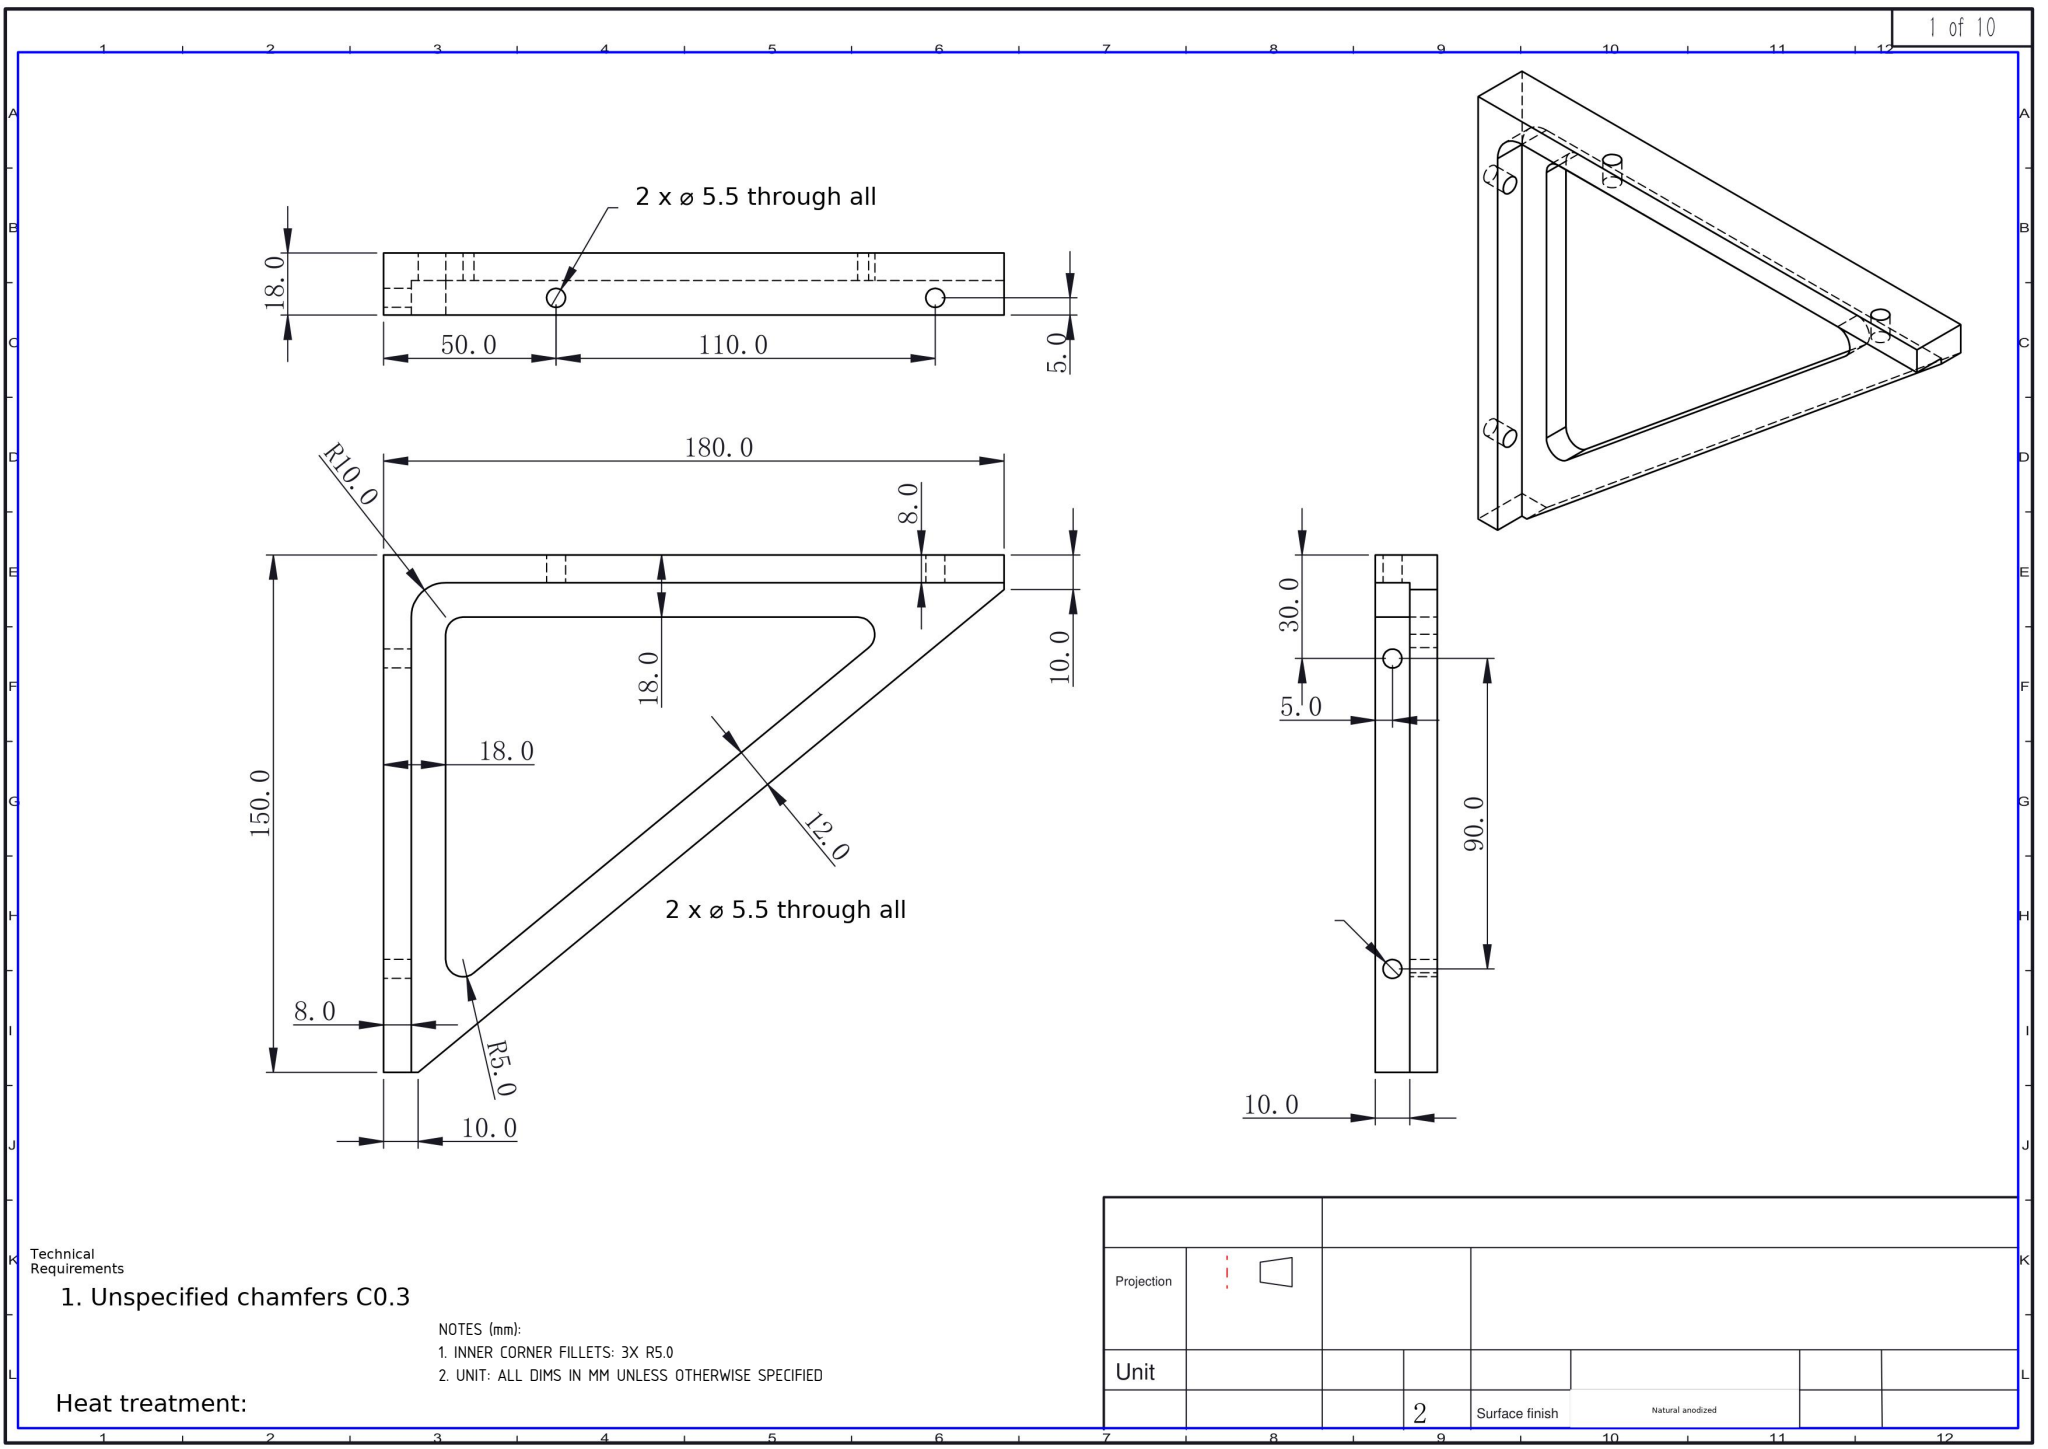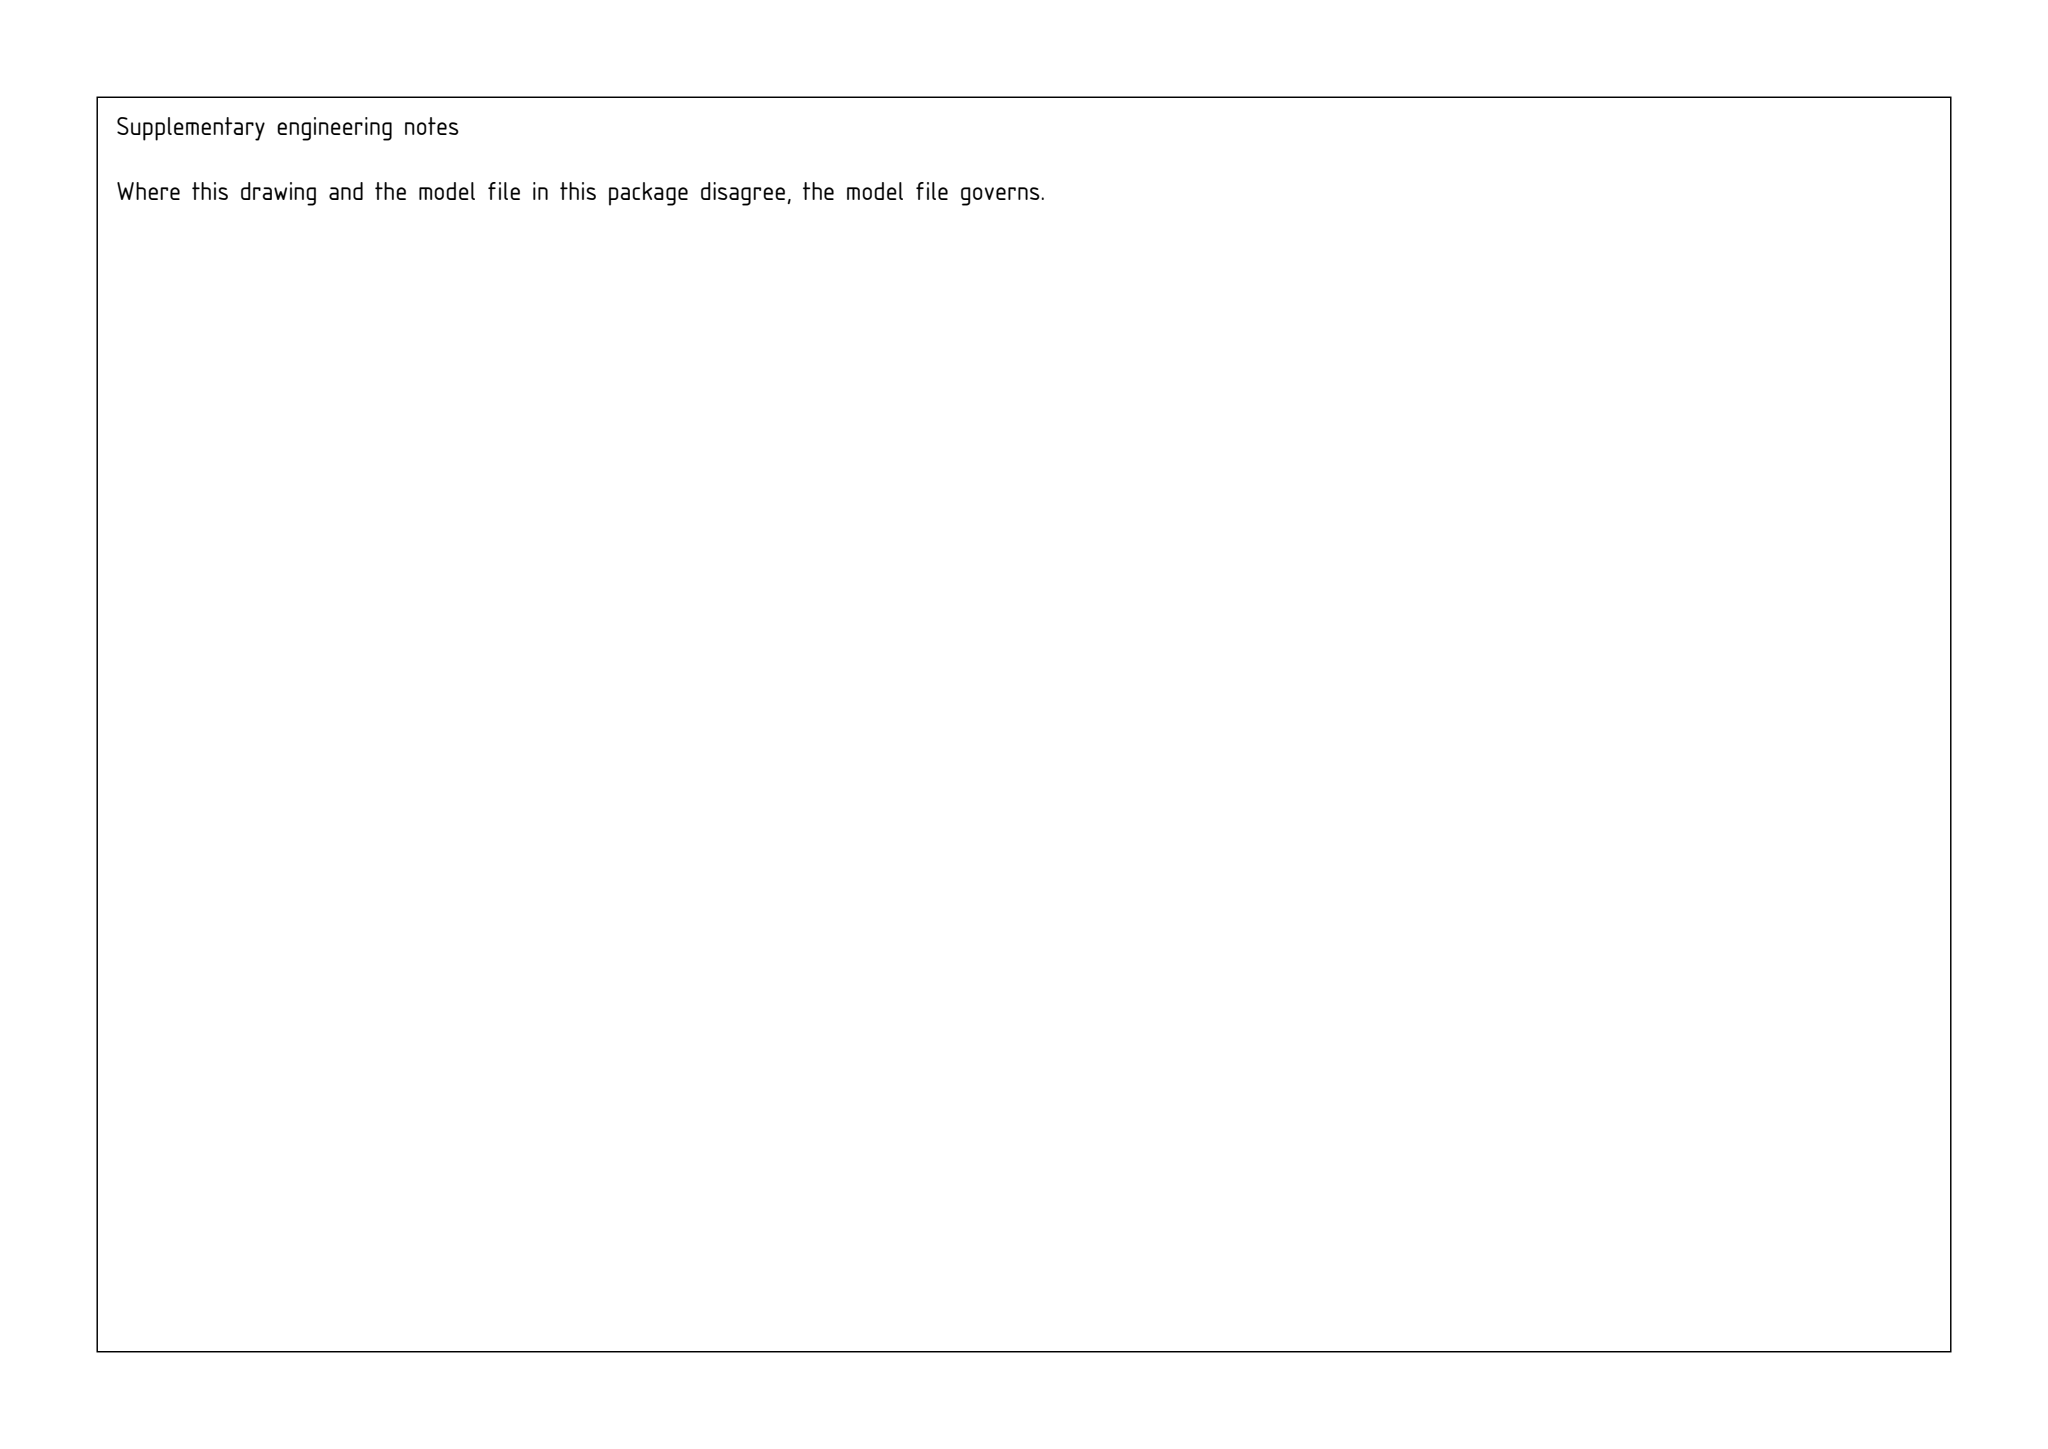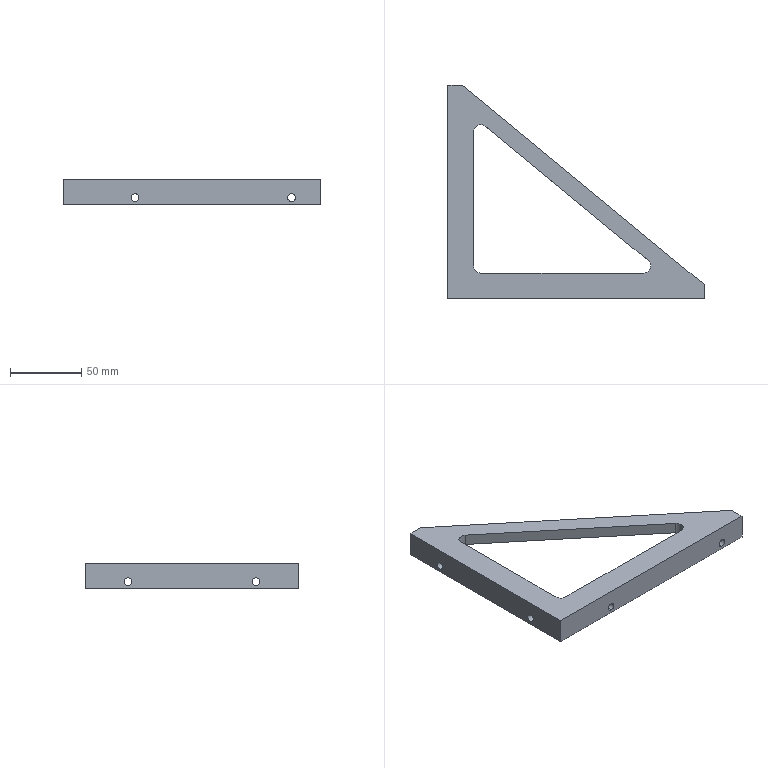Part | SolidWorks | mm | 1 solid | 25 faces | box 180 x 150 x 18 mm | volume 87939 mm3 | plane 13 | cylinder 12 | commonest cylinder face diameters 5.5 x8 10 x3 20 x1
Drawing notes:
INNER CORNER FILLETS: 3X R5.0 | from the solid: Three Ø10 z-axis cyls at (23,23), (23,117.27), (137.47,23) = R5.0 each
UNIT: ALL DIMS IN MM UNLESS OTHERWISE SPECIFIED | from the solid: STEP model bbox 180.0 x 150.0 x 18.0 mm matches drawing values
build123d program:
from build123d import *

# Parameters (mm, degrees)
BOSS_EXTRUDE1_DEPTH  = 18
CUT_EXTRUDE2_DEPTH   = 10
CUT_EXTRUDE3_DEPTH   = 235.521
M5_CLEARANCE_HOLE1_D = 5.5
M5_CLEARANCE_HOLE2_D = 5.5


with BuildPart() as part:
    # Sketch1 → Boss-Extrude1 (new body)
    with BuildSketch(Plane.XY):
        Polygon((10, 150), (180, 10), (180, 0), (0, 0), (0, 150), align=None)
    extrude(amount=BOSS_EXTRUDE1_DEPTH)

    # Sketch10 → Cut-Extrude2 (cut)
    with BuildSketch(Plane(origin=(0, 0, 0), x_dir=(-1, 0, 0), z_dir=(0, 0, -1))):
        with BuildLine():
            Line((-8, 150), (-180, 150))
            Line((-180, 150), (-180, 8))
            Line((-180, 8), (-18, 8))
            ThreePointArc((-18, 8), (-10.929, 10.929), (-8, 18))
            Line((-8, 18), (-8, 150))
        make_face()
    extrude(amount=-CUT_EXTRUDE2_DEPTH, mode=Mode.SUBTRACT)

    # Sketch11 → Cut-Extrude3 (cut, through all)
    with BuildSketch(Plane(origin=(0, 0, 10), x_dir=(-1, 0, 0), z_dir=(0, 0, -1))):
        with BuildLine():
            Line((-18, 23), (-18, 117.271))
            ThreePointArc((-18, 117.271), (-20.866, 121.793), (-26.179, 121.131))
            Line((-26.179, 121.131), (-140.651, 26.86))
            ThreePointArc((-140.651, 26.86), (-142.179, 21.312), (-137.472, 18))
            Line((-137.472, 18), (-23, 18))
            ThreePointArc((-23, 18), (-19.464, 19.464), (-18, 23))
        make_face()
    extrude(amount=-CUT_EXTRUDE3_DEPTH, mode=Mode.SUBTRACT)

    # M5 Clearance Hole1 (through all)
    with Locations(Plane(origin=(8, 0, 0), x_dir=(0, 0, -1), z_dir=(1, 0, 0))):
        with Locations((-5, 30), (-5, 120)):
            Hole(M5_CLEARANCE_HOLE1_D / 2)

    # M5 Clearance Hole2 (through all)
    with Locations(Plane(origin=(0, 8, 0), x_dir=(1, 0, 0), z_dir=(0, 1, 0))):
        with Locations((50, -5), (160, -5)):
            Hole(M5_CLEARANCE_HOLE2_D / 2)


solid = part.part
STEP:
#1=CARTESIAN_POINT('',(50.,-0.,2.25));
#2=VERTEX_POINT('',#1);
#3=CARTESIAN_POINT('',(50.,-0.,7.75));
#4=VERTEX_POINT('',#3);
#5=CARTESIAN_POINT('',(50.,-0.,5.));
#6=DIRECTION('',(0.,1.,0.));
#7=DIRECTION('',(0.,0.,1.));
#8=AXIS2_PLACEMENT_3D('',#5,#6,#7);
#9=CIRCLE('',#8,2.75);
#10=EDGE_CURVE('',#2,#4,#9,.T.);
#11=ORIENTED_EDGE('',*,*,#10,.F.);
#12=CARTESIAN_POINT('',(50.,8.,2.25));
#13=VERTEX_POINT('',#12);
#14=CARTESIAN_POINT('',(50.,8.,2.25));
#15=DIRECTION('',(0.,1.,0.));
#16=VECTOR('',#15,1000.);
#17=LINE('',#14,#16);
#18=EDGE_CURVE('',#2,#13,#17,.T.);
#19=ORIENTED_EDGE('',*,*,#18,.T.);
#20=CARTESIAN_POINT('',(50.,8.,7.75));
#21=VERTEX_POINT('',#20);
#22=CARTESIAN_POINT('',(50.,8.,5.));
#23=DIRECTION('',(0.,1.,0.));
#24=DIRECTION('',(0.,0.,1.));
#25=AXIS2_PLACEMENT_3D('',#22,#23,#24);
#26=CIRCLE('',#25,2.75);
#27=EDGE_CURVE('',#13,#21,#26,.T.);
#28=ORIENTED_EDGE('',*,*,#27,.T.);
#29=CARTESIAN_POINT('',(50.,8.,7.75));
#30=DIRECTION('',(0.,1.,0.));
#31=VECTOR('',#30,1000.);
#32=LINE('',#29,#31);
#33=EDGE_CURVE('',#4,#21,#32,.T.);
#34=ORIENTED_EDGE('',*,*,#33,.F.);
#35=EDGE_LOOP('',(#11,#19,#28,#34));
#36=FACE_OUTER_BOUND('',#35,.T.);
#37=CARTESIAN_POINT('',(50.,8.,5.));
#38=DIRECTION('',(0.,1.,0.));
#39=DIRECTION('',(0.,0.,1.));
#40=AXIS2_PLACEMENT_3D('',#37,#38,#39);
#41=CYLINDRICAL_SURFACE('',#40,2.75);
#42=ADVANCED_FACE('',(#36),#41,.F.);
#43=CARTESIAN_POINT('',(160.,-0.,2.25));
#44=VERTEX_POINT('',#43);
#45=CARTESIAN_POINT('',(160.,-0.,7.75));
#46=VERTEX_POINT('',#45);
#47=CARTESIAN_POINT('',(160.,-0.,5.));
#48=DIRECTION('',(0.,1.,0.));
#49=DIRECTION('',(0.,0.,1.));
#50=AXIS2_PLACEMENT_3D('',#47,#48,#49);
#51=CIRCLE('',#50,2.75);
#52=EDGE_CURVE('',#44,#46,#51,.T.);
#53=ORIENTED_EDGE('',*,*,#52,.F.);
#54=CARTESIAN_POINT('',(160.,8.,2.25));
#55=VERTEX_POINT('',#54);
#56=CARTESIAN_POINT('',(160.,8.,2.25));
#57=DIRECTION('',(0.,1.,0.));
#58=VECTOR('',#57,1000.);
#59=LINE('',#56,#58);
#60=EDGE_CURVE('',#44,#55,#59,.T.);
#61=ORIENTED_EDGE('',*,*,#60,.T.);
#62=CARTESIAN_POINT('',(160.,8.,7.75));
#63=VERTEX_POINT('',#62);
#64=CARTESIAN_POINT('',(160.,8.,5.));
#65=DIRECTION('',(0.,1.,0.));
#66=DIRECTION('',(0.,0.,1.));
#67=AXIS2_PLACEMENT_3D('',#64,#65,#66);
#68=CIRCLE('',#67,2.75);
#69=EDGE_CURVE('',#55,#63,#68,.T.);
#70=ORIENTED_EDGE('',*,*,#69,.T.);
#71=CARTESIAN_POINT('',(160.,8.,7.75));
#72=DIRECTION('',(0.,1.,0.));
#73=VECTOR('',#72,1000.);
#74=LINE('',#71,#73);
#75=EDGE_CURVE('',#46,#63,#74,.T.);
#76=ORIENTED_EDGE('',*,*,#75,.F.);
#77=EDGE_LOOP('',(#53,#61,#70,#76));
#78=FACE_OUTER_BOUND('',#77,.T.);
#79=CARTESIAN_POINT('',(160.,8.,5.));
#80=DIRECTION('',(0.,1.,0.));
#81=DIRECTION('',(0.,0.,1.));
#82=AXIS2_PLACEMENT_3D('',#79,#80,#81);
#83=CYLINDRICAL_SURFACE('',#82,2.75);
#84=ADVANCED_FACE('',(#78),#83,.F.);
#85=CARTESIAN_POINT('',(-0.,30.,7.75));
#86=VERTEX_POINT('',#85);
#87=CARTESIAN_POINT('',(-0.,30.,2.25));
#88=VERTEX_POINT('',#87);
#89=CARTESIAN_POINT('',(-0.,30.,5.));
#90=DIRECTION('',(1.,0.,0.));
#91=DIRECTION('',(0.,0.,-1.));
#92=AXIS2_PLACEMENT_3D('',#89,#90,#91);
#93=CIRCLE('',#92,2.75);
#94=EDGE_CURVE('',#86,#88,#93,.T.);
#95=ORIENTED_EDGE('',*,*,#94,.F.);
#96=CARTESIAN_POINT('',(8.,30.,7.75));
#97=VERTEX_POINT('',#96);
#98=CARTESIAN_POINT('',(8.,30.,7.75));
#99=DIRECTION('',(1.,0.,0.));
#100=VECTOR('',#99,1000.);
#101=LINE('',#98,#100);
#102=EDGE_CURVE('',#86,#97,#101,.T.);
#103=ORIENTED_EDGE('',*,*,#102,.T.);
#104=CARTESIAN_POINT('',(8.,30.,2.25));
#105=VERTEX_POINT('',#104);
#106=CARTESIAN_POINT('',(8.,30.,5.));
#107=DIRECTION('',(1.,0.,0.));
#108=DIRECTION('',(0.,0.,-1.));
#109=AXIS2_PLACEMENT_3D('',#106,#107,#108);
#110=CIRCLE('',#109,2.75);
#111=EDGE_CURVE('',#97,#105,#110,.T.);
#112=ORIENTED_EDGE('',*,*,#111,.T.);
#113=CARTESIAN_POINT('',(8.,30.,2.25));
#114=DIRECTION('',(1.,0.,0.));
#115=VECTOR('',#114,1000.);
#116=LINE('',#113,#115);
#117=EDGE_CURVE('',#88,#105,#116,.T.);
#118=ORIENTED_EDGE('',*,*,#117,.F.);
#119=EDGE_LOOP('',(#95,#103,#112,#118));
#120=FACE_OUTER_BOUND('',#119,.T.);
#121=CARTESIAN_POINT('',(8.,30.,5.));
#122=DIRECTION('',(1.,0.,0.));
#123=DIRECTION('',(0.,0.,-1.));
#124=AXIS2_PLACEMENT_3D('',#121,#122,#123);
#125=CYLINDRICAL_SURFACE('',#124,2.75);
#126=ADVANCED_FACE('',(#120),#125,.F.);
#127=CARTESIAN_POINT('',(-0.,120.,7.75));
#128=VERTEX_POINT('',#127);
#129=CARTESIAN_POINT('',(-0.,120.,2.25));
#130=VERTEX_POINT('',#129);
#131=CARTESIAN_POINT('',(-0.,120.,5.));
#132=DIRECTION('',(1.,0.,0.));
#133=DIRECTION('',(0.,0.,-1.));
#134=AXIS2_PLACEMENT_3D('',#131,#132,#133);
#135=CIRCLE('',#134,2.75);
#136=EDGE_CURVE('',#128,#130,#135,.T.);
#137=ORIENTED_EDGE('',*,*,#136,.F.);
#138=CARTESIAN_POINT('',(8.,120.,7.75));
#139=VERTEX_POINT('',#138);
#140=CARTESIAN_POINT('',(8.,120.,7.75));
#141=DIRECTION('',(1.,0.,0.));
#142=VECTOR('',#141,1000.);
#143=LINE('',#140,#142);
#144=EDGE_CURVE('',#128,#139,#143,.T.);
#145=ORIENTED_EDGE('',*,*,#144,.T.);
#146=CARTESIAN_POINT('',(8.,120.,2.25));
#147=VERTEX_POINT('',#146);
#148=CARTESIAN_POINT('',(8.,120.,5.));
#149=DIRECTION('',(1.,0.,0.));
#150=DIRECTION('',(0.,0.,-1.));
#151=AXIS2_PLACEMENT_3D('',#148,#149,#150);
#152=CIRCLE('',#151,2.75);
#153=EDGE_CURVE('',#139,#147,#152,.T.);
#154=ORIENTED_EDGE('',*,*,#153,.T.);
#155=CARTESIAN_POINT('',(8.,120.,2.25));
#156=DIRECTION('',(1.,0.,0.));
#157=VECTOR('',#156,1000.);
#158=LINE('',#155,#157);
#159=EDGE_CURVE('',#130,#147,#158,.T.);
#160=ORIENTED_EDGE('',*,*,#159,.F.);
#161=EDGE_LOOP('',(#137,#145,#154,#160));
#162=FACE_OUTER_BOUND('',#161,.T.);
#163=CARTESIAN_POINT('',(8.,120.,5.));
#164=DIRECTION('',(1.,0.,0.));
#165=DIRECTION('',(0.,0.,-1.));
#166=AXIS2_PLACEMENT_3D('',#163,#164,#165);
#167=CYLINDRICAL_SURFACE('',#166,2.75);
#168=ADVANCED_FACE('',(#162),#167,.F.);
#169=CARTESIAN_POINT('',(-0.,30.,5.));
#170=DIRECTION('',(1.,0.,0.));
#171=DIRECTION('',(0.,0.,-1.));
#172=AXIS2_PLACEMENT_3D('',#169,#170,#171);
#173=CIRCLE('',#172,2.75);
#174=EDGE_CURVE('',#88,#86,#173,.T.);
#175=ORIENTED_EDGE('',*,*,#174,.T.);
#176=ORIENTED_EDGE('',*,*,#94,.T.);
#177=EDGE_LOOP('',(#175,#176));
#178=FACE_BOUND('',#177,.T.);
#179=CARTESIAN_POINT('',(-0.,120.,5.));
#180=DIRECTION('',(1.,0.,0.));
#181=DIRECTION('',(0.,0.,-1.));
#182=AXIS2_PLACEMENT_3D('',#179,#180,#181);
#183=CIRCLE('',#182,2.75);
#184=EDGE_CURVE('',#130,#128,#183,.T.);
#185=ORIENTED_EDGE('',*,*,#184,.T.);
#186=ORIENTED_EDGE('',*,*,#136,.T.);
#187=EDGE_LOOP('',(#185,#186));
#188=FACE_BOUND('',#187,.T.);
#189=CARTESIAN_POINT('',(0.,150.,0.));
#190=VERTEX_POINT('',#189);
#191=CARTESIAN_POINT('',(0.,0.,0.));
#192=VERTEX_POINT('',#191);
#193=CARTESIAN_POINT('',(0.,0.,0.));
#194=DIRECTION('',(0.,-1.,0.));
#195=VECTOR('',#194,1000.);
#196=LINE('',#193,#195);
#197=EDGE_CURVE('',#190,#192,#196,.T.);
#198=ORIENTED_EDGE('',*,*,#197,.T.);
#199=CARTESIAN_POINT('',(0.,0.,18.));
#200=VERTEX_POINT('',#199);
#201=CARTESIAN_POINT('',(0.,0.,18.));
#202=DIRECTION('',(0.,0.,-1.));
#203=VECTOR('',#202,1000.);
#204=LINE('',#201,#203);
#205=EDGE_CURVE('',#200,#192,#204,.T.);
#206=ORIENTED_EDGE('',*,*,#205,.F.);
#207=CARTESIAN_POINT('',(0.,150.,18.));
#208=VERTEX_POINT('',#207);
#209=CARTESIAN_POINT('',(0.,0.,18.));
#210=DIRECTION('',(0.,-1.,0.));
#211=VECTOR('',#210,1000.);
#212=LINE('',#209,#211);
#213=EDGE_CURVE('',#208,#200,#212,.T.);
#214=ORIENTED_EDGE('',*,*,#213,.F.);
#215=CARTESIAN_POINT('',(0.,150.,18.));
#216=DIRECTION('',(0.,0.,-1.));
#217=VECTOR('',#216,1000.);
#218=LINE('',#215,#217);
#219=EDGE_CURVE('',#208,#190,#218,.T.);
#220=ORIENTED_EDGE('',*,*,#219,.T.);
#221=EDGE_LOOP('',(#198,#206,#214,#220));
#222=FACE_OUTER_BOUND('',#221,.T.);
#223=CARTESIAN_POINT('',(0.,0.,18.));
#224=DIRECTION('',(1.,0.,0.));
#225=DIRECTION('',(0.,0.,-1.));
#226=AXIS2_PLACEMENT_3D('',#223,#224,#225);
#227=PLANE('',#226);
#228=ADVANCED_FACE('',(#178,#188,#222),#227,.F.);
#229=CARTESIAN_POINT('',(50.,-0.,5.));
#230=DIRECTION('',(0.,1.,0.));
#231=DIRECTION('',(0.,0.,1.));
#232=AXIS2_PLACEMENT_3D('',#229,#230,#231);
#233=CIRCLE('',#232,2.75);
#234=EDGE_CURVE('',#4,#2,#233,.T.);
#235=ORIENTED_EDGE('',*,*,#234,.T.);
#236=ORIENTED_EDGE('',*,*,#10,.T.);
#237=EDGE_LOOP('',(#235,#236));
#238=FACE_BOUND('',#237,.T.);
#239=CARTESIAN_POINT('',(160.,-0.,5.));
#240=DIRECTION('',(0.,1.,0.));
#241=DIRECTION('',(0.,0.,1.));
#242=AXIS2_PLACEMENT_3D('',#239,#240,#241);
#243=CIRCLE('',#242,2.75);
#244=EDGE_CURVE('',#46,#44,#243,.T.);
#245=ORIENTED_EDGE('',*,*,#244,.T.);
#246=ORIENTED_EDGE('',*,*,#52,.T.);
#247=EDGE_LOOP('',(#245,#246));
#248=FACE_BOUND('',#247,.T.);
#249=CARTESIAN_POINT('',(180.,0.,0.));
#250=VERTEX_POINT('',#249);
#251=CARTESIAN_POINT('',(0.,0.,0.));
#252=DIRECTION('',(1.,0.,0.));
#253=VECTOR('',#252,1000.);
#254=LINE('',#251,#253);
#255=EDGE_CURVE('',#192,#250,#254,.T.);
#256=ORIENTED_EDGE('',*,*,#255,.T.);
#257=CARTESIAN_POINT('',(180.,0.,18.));
#258=VERTEX_POINT('',#257);
#259=CARTESIAN_POINT('',(180.,0.,18.));
#260=DIRECTION('',(0.,0.,-1.));
#261=VECTOR('',#260,1000.);
#262=LINE('',#259,#261);
#263=EDGE_CURVE('',#258,#250,#262,.T.);
#264=ORIENTED_EDGE('',*,*,#263,.F.);
#265=CARTESIAN_POINT('',(0.,0.,18.));
#266=DIRECTION('',(1.,0.,0.));
#267=VECTOR('',#266,1000.);
#268=LINE('',#265,#267);
#269=EDGE_CURVE('',#200,#258,#268,.T.);
#270=ORIENTED_EDGE('',*,*,#269,.F.);
#271=ORIENTED_EDGE('',*,*,#205,.T.);
#272=EDGE_LOOP('',(#256,#264,#270,#271));
#273=FACE_OUTER_BOUND('',#272,.T.);
#274=CARTESIAN_POINT('',(0.,0.,18.));
#275=DIRECTION('',(0.,1.,0.));
#276=DIRECTION('',(0.,0.,1.));
#277=AXIS2_PLACEMENT_3D('',#274,#275,#276);
#278=PLANE('',#277);
#279=ADVANCED_FACE('',(#238,#248,#273),#278,.F.);
#280=CARTESIAN_POINT('',(180.,8.,0.));
#281=VERTEX_POINT('',#280);
#282=CARTESIAN_POINT('',(180.,0.,0.));
#283=DIRECTION('',(0.,1.,0.));
#284=VECTOR('',#283,1000.);
#285=LINE('',#282,#284);
#286=EDGE_CURVE('',#250,#281,#285,.T.);
#287=ORIENTED_EDGE('',*,*,#286,.T.);
#288=CARTESIAN_POINT('',(180.,8.,10.));
#289=VERTEX_POINT('',#288);
#290=CARTESIAN_POINT('',(180.,8.,10.));
#291=DIRECTION('',(0.,0.,-1.));
#292=VECTOR('',#291,1000.);
#293=LINE('',#290,#292);
#294=EDGE_CURVE('',#289,#281,#293,.T.);
#295=ORIENTED_EDGE('',*,*,#294,.F.);
#296=CARTESIAN_POINT('',(180.,10.,10.));
#297=VERTEX_POINT('',#296);
#298=CARTESIAN_POINT('',(180.,150.,10.));
#299=DIRECTION('',(0.,-1.,0.));
#300=VECTOR('',#299,1000.);
#301=LINE('',#298,#300);
#302=EDGE_CURVE('',#297,#289,#301,.T.);
#303=ORIENTED_EDGE('',*,*,#302,.F.);
#304=CARTESIAN_POINT('',(180.,10.,18.));
#305=VERTEX_POINT('',#304);
#306=CARTESIAN_POINT('',(180.,10.,18.));
#307=DIRECTION('',(0.,0.,-1.));
#308=VECTOR('',#307,1000.);
#309=LINE('',#306,#308);
#310=EDGE_CURVE('',#305,#297,#309,.T.);
#311=ORIENTED_EDGE('',*,*,#310,.F.);
#312=CARTESIAN_POINT('',(180.,0.,18.));
#313=DIRECTION('',(0.,1.,0.));
#314=VECTOR('',#313,1000.);
#315=LINE('',#312,#314);
#316=EDGE_CURVE('',#258,#305,#315,.T.);
#317=ORIENTED_EDGE('',*,*,#316,.F.);
#318=ORIENTED_EDGE('',*,*,#263,.T.);
#319=EDGE_LOOP('',(#287,#295,#303,#311,#317,#318));
#320=FACE_OUTER_BOUND('',#319,.T.);
#321=CARTESIAN_POINT('',(180.,0.,18.));
#322=DIRECTION('',(-1.,0.,0.));
#323=DIRECTION('',(0.,0.,1.));
#324=AXIS2_PLACEMENT_3D('',#321,#322,#323);
#325=PLANE('',#324);
#326=ADVANCED_FACE('',(#320),#325,.F.);
#327=ORIENTED_EDGE('',*,*,#310,.T.);
#328=CARTESIAN_POINT('',(10.,150.,10.));
#329=VERTEX_POINT('',#328);
#330=CARTESIAN_POINT('',(10.,150.,10.));
#331=DIRECTION('',(-0.7719,0.6357,0.));
#332=VECTOR('',#331,1000.);
#333=LINE('',#330,#332);
#334=EDGE_CURVE('',#297,#329,#333,.T.);
#335=ORIENTED_EDGE('',*,*,#334,.T.);
#336=CARTESIAN_POINT('',(10.,150.,18.));
#337=VERTEX_POINT('',#336);
#338=CARTESIAN_POINT('',(10.,150.,18.));
#339=DIRECTION('',(0.,0.,-1.));
#340=VECTOR('',#339,1000.);
#341=LINE('',#338,#340);
#342=EDGE_CURVE('',#337,#329,#341,.T.);
#343=ORIENTED_EDGE('',*,*,#342,.F.);
#344=CARTESIAN_POINT('',(10.,150.,18.));
#345=DIRECTION('',(-0.7719,0.6357,0.));
#346=VECTOR('',#345,1000.);
#347=LINE('',#344,#346);
#348=EDGE_CURVE('',#305,#337,#347,.T.);
#349=ORIENTED_EDGE('',*,*,#348,.F.);
#350=EDGE_LOOP('',(#327,#335,#343,#349));
#351=FACE_OUTER_BOUND('',#350,.T.);
#352=CARTESIAN_POINT('',(10.,150.,18.));
#353=DIRECTION('',(-0.6357,-0.7719,0.));
#354=DIRECTION('',(0.7719,-0.6357,0.));
#355=AXIS2_PLACEMENT_3D('',#352,#353,#354);
#356=PLANE('',#355);
#357=ADVANCED_FACE('',(#351),#356,.F.);
#358=CARTESIAN_POINT('',(8.,150.,10.));
#359=VERTEX_POINT('',#358);
#360=CARTESIAN_POINT('',(8.,150.,10.));
#361=DIRECTION('',(1.,0.,0.));
#362=VECTOR('',#361,1000.);
#363=LINE('',#360,#362);
#364=EDGE_CURVE('',#359,#329,#363,.T.);
#365=ORIENTED_EDGE('',*,*,#364,.F.);
#366=CARTESIAN_POINT('',(8.,150.,0.));
#367=VERTEX_POINT('',#366);
#368=CARTESIAN_POINT('',(8.,150.,10.));
#369=DIRECTION('',(0.,0.,-1.));
#370=VECTOR('',#369,1000.);
#371=LINE('',#368,#370);
#372=EDGE_CURVE('',#359,#367,#371,.T.);
#373=ORIENTED_EDGE('',*,*,#372,.T.);
#374=CARTESIAN_POINT('',(0.,150.,0.));
#375=DIRECTION('',(-1.,0.,0.));
#376=VECTOR('',#375,1000.);
#377=LINE('',#374,#376);
#378=EDGE_CURVE('',#367,#190,#377,.T.);
#379=ORIENTED_EDGE('',*,*,#378,.T.);
#380=ORIENTED_EDGE('',*,*,#219,.F.);
#381=CARTESIAN_POINT('',(0.,150.,18.));
#382=DIRECTION('',(-1.,0.,0.));
#383=VECTOR('',#382,1000.);
#384=LINE('',#381,#383);
#385=EDGE_CURVE('',#337,#208,#384,.T.);
#386=ORIENTED_EDGE('',*,*,#385,.F.);
#387=ORIENTED_EDGE('',*,*,#342,.T.);
#388=EDGE_LOOP('',(#365,#373,#379,#380,#386,#387));
#389=FACE_OUTER_BOUND('',#388,.T.);
#390=CARTESIAN_POINT('',(0.,150.,18.));
#391=DIRECTION('',(0.,-1.,0.));
#392=DIRECTION('',(0.,0.,-1.));
#393=AXIS2_PLACEMENT_3D('',#390,#391,#392);
#394=PLANE('',#393);
#395=ADVANCED_FACE('',(#389),#394,.F.);
#396=CARTESIAN_POINT('',(137.472,18.,18.));
#397=VERTEX_POINT('',#396);
#398=CARTESIAN_POINT('',(23.,18.,18.));
#399=VERTEX_POINT('',#398);
#400=CARTESIAN_POINT('',(137.472,18.,18.));
#401=DIRECTION('',(-1.,0.,0.));
#402=VECTOR('',#401,1000.);
#403=LINE('',#400,#402);
#404=EDGE_CURVE('',#397,#399,#403,.T.);
#405=ORIENTED_EDGE('',*,*,#404,.T.);
#406=CARTESIAN_POINT('',(18.,23.,18.));
#407=VERTEX_POINT('',#406);
#408=CARTESIAN_POINT('',(23.,23.,18.));
#409=DIRECTION('',(0.,0.,-1.));
#410=DIRECTION('',(1.,0.,0.));
#411=AXIS2_PLACEMENT_3D('',#408,#409,#410);
#412=CIRCLE('',#411,5.);
#413=EDGE_CURVE('',#399,#407,#412,.T.);
#414=ORIENTED_EDGE('',*,*,#413,.T.);
#415=CARTESIAN_POINT('',(18.,117.271,18.));
#416=VERTEX_POINT('',#415);
#417=CARTESIAN_POINT('',(18.,23.,18.));
#418=DIRECTION('',(-0.,1.,0.));
#419=VECTOR('',#418,1000.);
#420=LINE('',#417,#419);
#421=EDGE_CURVE('',#407,#416,#420,.T.);
#422=ORIENTED_EDGE('',*,*,#421,.T.);
#423=CARTESIAN_POINT('',(26.179,121.131,18.));
#424=VERTEX_POINT('',#423);
#425=CARTESIAN_POINT('',(23.,117.271,18.));
#426=DIRECTION('',(0.,0.,-1.));
#427=DIRECTION('',(-1.,0.,0.));
#428=AXIS2_PLACEMENT_3D('',#425,#426,#427);
#429=CIRCLE('',#428,5.);
#430=EDGE_CURVE('',#416,#424,#429,.T.);
#431=ORIENTED_EDGE('',*,*,#430,.T.);
#432=CARTESIAN_POINT('',(140.651,26.86,18.));
#433=VERTEX_POINT('',#432);
#434=CARTESIAN_POINT('',(26.179,121.131,18.));
#435=DIRECTION('',(0.7719,-0.6357,0.));
#436=VECTOR('',#435,1000.);
#437=LINE('',#434,#436);
#438=EDGE_CURVE('',#424,#433,#437,.T.);
#439=ORIENTED_EDGE('',*,*,#438,.T.);
#440=CARTESIAN_POINT('',(137.472,23.,18.));
#441=DIRECTION('',(0.,0.,-1.));
#442=DIRECTION('',(-1.,0.,0.));
#443=AXIS2_PLACEMENT_3D('',#440,#441,#442);
#444=CIRCLE('',#443,5.);
#445=EDGE_CURVE('',#433,#397,#444,.T.);
#446=ORIENTED_EDGE('',*,*,#445,.T.);
#447=EDGE_LOOP('',(#405,#414,#422,#431,#439,#446));
#448=FACE_BOUND('',#447,.T.);
#449=ORIENTED_EDGE('',*,*,#213,.T.);
#450=ORIENTED_EDGE('',*,*,#269,.T.);
#451=ORIENTED_EDGE('',*,*,#316,.T.);
#452=ORIENTED_EDGE('',*,*,#348,.T.);
#453=ORIENTED_EDGE('',*,*,#385,.T.);
#454=EDGE_LOOP('',(#449,#450,#451,#452,#453));
#455=FACE_OUTER_BOUND('',#454,.T.);
#456=CARTESIAN_POINT('',(0.,0.,18.));
#457=DIRECTION('',(0.,0.,-1.));
#458=DIRECTION('',(-1.,0.,0.));
#459=AXIS2_PLACEMENT_3D('',#456,#457,#458);
#460=PLANE('',#459);
#461=ADVANCED_FACE('',(#448,#455),#460,.F.);
#462=CARTESIAN_POINT('',(8.,18.,0.));
#463=VERTEX_POINT('',#462);
#464=CARTESIAN_POINT('',(8.,150.,0.));
#465=DIRECTION('',(0.,1.,0.));
#466=VECTOR('',#465,1000.);
#467=LINE('',#464,#466);
#468=EDGE_CURVE('',#463,#367,#467,.T.);
#469=ORIENTED_EDGE('',*,*,#468,.F.);
#470=CARTESIAN_POINT('',(18.,8.,0.));
#471=VERTEX_POINT('',#470);
#472=CARTESIAN_POINT('',(18.,18.,0.));
#473=DIRECTION('',(0.,0.,-1.));
#474=DIRECTION('',(1.,0.,0.));
#475=AXIS2_PLACEMENT_3D('',#472,#473,#474);
#476=CIRCLE('',#475,10.);
#477=EDGE_CURVE('',#471,#463,#476,.T.);
#478=ORIENTED_EDGE('',*,*,#477,.F.);
#479=CARTESIAN_POINT('',(18.,8.,0.));
#480=DIRECTION('',(-1.,0.,0.));
#481=VECTOR('',#480,1000.);
#482=LINE('',#479,#481);
#483=EDGE_CURVE('',#281,#471,#482,.T.);
#484=ORIENTED_EDGE('',*,*,#483,.F.);
#485=ORIENTED_EDGE('',*,*,#286,.F.);
#486=ORIENTED_EDGE('',*,*,#255,.F.);
#487=ORIENTED_EDGE('',*,*,#197,.F.);
#488=ORIENTED_EDGE('',*,*,#378,.F.);
#489=EDGE_LOOP('',(#469,#478,#484,#485,#486,#487,#488));
#490=FACE_OUTER_BOUND('',#489,.T.);
#491=CARTESIAN_POINT('',(0.,0.,0.));
#492=DIRECTION('',(0.,0.,-1.));
#493=DIRECTION('',(-1.,0.,0.));
#494=AXIS2_PLACEMENT_3D('',#491,#492,#493);
#495=PLANE('',#494);
#496=ADVANCED_FACE('',(#490),#495,.T.);
#497=CARTESIAN_POINT('',(18.,23.,10.));
#498=VERTEX_POINT('',#497);
#499=CARTESIAN_POINT('',(18.,117.271,10.));
#500=VERTEX_POINT('',#499);
#501=CARTESIAN_POINT('',(18.,23.,10.));
#502=DIRECTION('',(-0.,1.,0.));
#503=VECTOR('',#502,1000.);
#504=LINE('',#501,#503);
#505=EDGE_CURVE('',#498,#500,#504,.T.);
#506=ORIENTED_EDGE('',*,*,#505,.F.);
#507=CARTESIAN_POINT('',(23.,18.,10.));
#508=VERTEX_POINT('',#507);
#509=CARTESIAN_POINT('',(23.,23.,10.));
#510=DIRECTION('',(0.,0.,-1.));
#511=DIRECTION('',(1.,0.,0.));
#512=AXIS2_PLACEMENT_3D('',#509,#510,#511);
#513=CIRCLE('',#512,5.);
#514=EDGE_CURVE('',#508,#498,#513,.T.);
#515=ORIENTED_EDGE('',*,*,#514,.F.);
#516=CARTESIAN_POINT('',(137.472,18.,10.));
#517=VERTEX_POINT('',#516);
#518=CARTESIAN_POINT('',(137.472,18.,10.));
#519=DIRECTION('',(-1.,0.,0.));
#520=VECTOR('',#519,1000.);
#521=LINE('',#518,#520);
#522=EDGE_CURVE('',#517,#508,#521,.T.);
#523=ORIENTED_EDGE('',*,*,#522,.F.);
#524=CARTESIAN_POINT('',(140.651,26.86,10.));
#525=VERTEX_POINT('',#524);
#526=CARTESIAN_POINT('',(137.472,23.,10.));
#527=DIRECTION('',(0.,0.,-1.));
#528=DIRECTION('',(-1.,0.,0.));
#529=AXIS2_PLACEMENT_3D('',#526,#527,#528);
#530=CIRCLE('',#529,5.);
#531=EDGE_CURVE('',#525,#517,#530,.T.);
#532=ORIENTED_EDGE('',*,*,#531,.F.);
#533=CARTESIAN_POINT('',(26.179,121.131,10.));
#534=VERTEX_POINT('',#533);
#535=CARTESIAN_POINT('',(26.179,121.131,10.));
#536=DIRECTION('',(0.7719,-0.6357,0.));
#537=VECTOR('',#536,1000.);
#538=LINE('',#535,#537);
#539=EDGE_CURVE('',#534,#525,#538,.T.);
#540=ORIENTED_EDGE('',*,*,#539,.F.);
#541=CARTESIAN_POINT('',(23.,117.271,10.));
#542=DIRECTION('',(0.,0.,-1.));
#543=DIRECTION('',(-1.,0.,0.));
#544=AXIS2_PLACEMENT_3D('',#541,#542,#543);
#545=CIRCLE('',#544,5.);
#546=EDGE_CURVE('',#500,#534,#545,.T.);
#547=ORIENTED_EDGE('',*,*,#546,.F.);
#548=EDGE_LOOP('',(#506,#515,#523,#532,#540,#547));
#549=FACE_BOUND('',#548,.T.);
#550=ORIENTED_EDGE('',*,*,#302,.T.);
#551=CARTESIAN_POINT('',(18.,8.,10.));
#552=VERTEX_POINT('',#551);
#553=CARTESIAN_POINT('',(18.,8.,10.));
#554=DIRECTION('',(-1.,0.,0.));
#555=VECTOR('',#554,1000.);
#556=LINE('',#553,#555);
#557=EDGE_CURVE('',#289,#552,#556,.T.);
#558=ORIENTED_EDGE('',*,*,#557,.T.);
#559=CARTESIAN_POINT('',(8.,18.,10.));
#560=VERTEX_POINT('',#559);
#561=CARTESIAN_POINT('',(18.,18.,10.));
#562=DIRECTION('',(0.,0.,-1.));
#563=DIRECTION('',(1.,0.,0.));
#564=AXIS2_PLACEMENT_3D('',#561,#562,#563);
#565=CIRCLE('',#564,10.);
#566=EDGE_CURVE('',#552,#560,#565,.T.);
#567=ORIENTED_EDGE('',*,*,#566,.T.);
#568=CARTESIAN_POINT('',(8.,150.,10.));
#569=DIRECTION('',(0.,1.,0.));
#570=VECTOR('',#569,1000.);
#571=LINE('',#568,#570);
#572=EDGE_CURVE('',#560,#359,#571,.T.);
#573=ORIENTED_EDGE('',*,*,#572,.T.);
#574=ORIENTED_EDGE('',*,*,#364,.T.);
#575=ORIENTED_EDGE('',*,*,#334,.F.);
#576=EDGE_LOOP('',(#550,#558,#567,#573,#574,#575));
#577=FACE_OUTER_BOUND('',#576,.T.);
#578=CARTESIAN_POINT('',(18.,18.,10.));
#579=DIRECTION('',(0.,0.,1.));
#580=DIRECTION('',(1.,0.,0.));
#581=AXIS2_PLACEMENT_3D('',#578,#579,#580);
#582=PLANE('',#581);
#583=ADVANCED_FACE('',(#549,#577),#582,.F.);
#584=CARTESIAN_POINT('',(8.,30.,5.));
#585=DIRECTION('',(1.,0.,0.));
#586=DIRECTION('',(0.,0.,-1.));
#587=AXIS2_PLACEMENT_3D('',#584,#585,#586);
#588=CIRCLE('',#587,2.75);
#589=EDGE_CURVE('',#105,#97,#588,.T.);
#590=ORIENTED_EDGE('',*,*,#589,.F.);
#591=ORIENTED_EDGE('',*,*,#111,.F.);
#592=EDGE_LOOP('',(#590,#591));
#593=FACE_BOUND('',#592,.T.);
#594=CARTESIAN_POINT('',(8.,120.,5.));
#595=DIRECTION('',(1.,0.,0.));
#596=DIRECTION('',(0.,0.,-1.));
#597=AXIS2_PLACEMENT_3D('',#594,#595,#596);
#598=CIRCLE('',#597,2.75);
#599=EDGE_CURVE('',#147,#139,#598,.T.);
#600=ORIENTED_EDGE('',*,*,#599,.F.);
#601=ORIENTED_EDGE('',*,*,#153,.F.);
#602=EDGE_LOOP('',(#600,#601));
#603=FACE_BOUND('',#602,.T.);
#604=ORIENTED_EDGE('',*,*,#468,.T.);
#605=ORIENTED_EDGE('',*,*,#372,.F.);
#606=ORIENTED_EDGE('',*,*,#572,.F.);
#607=CARTESIAN_POINT('',(8.,18.,10.));
#608=DIRECTION('',(0.,0.,-1.));
#609=VECTOR('',#608,1000.);
#610=LINE('',#607,#609);
#611=EDGE_CURVE('',#560,#463,#610,.T.);
#612=ORIENTED_EDGE('',*,*,#611,.T.);
#613=EDGE_LOOP('',(#604,#605,#606,#612));
#614=FACE_OUTER_BOUND('',#613,.T.);
#615=CARTESIAN_POINT('',(8.,150.,10.));
#616=DIRECTION('',(-1.,0.,0.));
#617=DIRECTION('',(-0.,-1.,0.));
#618=AXIS2_PLACEMENT_3D('',#615,#616,#617);
#619=PLANE('',#618);
#620=ADVANCED_FACE('',(#593,#603,#614),#619,.F.);
#621=ORIENTED_EDGE('',*,*,#477,.T.);
#622=ORIENTED_EDGE('',*,*,#611,.F.);
#623=ORIENTED_EDGE('',*,*,#566,.F.);
#624=CARTESIAN_POINT('',(18.,8.,10.));
#625=DIRECTION('',(0.,0.,-1.));
#626=VECTOR('',#625,1000.);
#627=LINE('',#624,#626);
#628=EDGE_CURVE('',#552,#471,#627,.T.);
#629=ORIENTED_EDGE('',*,*,#628,.T.);
#630=EDGE_LOOP('',(#621,#622,#623,#629));
#631=FACE_OUTER_BOUND('',#630,.T.);
#632=CARTESIAN_POINT('',(18.,18.,10.));
#633=DIRECTION('',(0.,0.,-1.));
#634=DIRECTION('',(-1.,0.,0.));
#635=AXIS2_PLACEMENT_3D('',#632,#633,#634);
#636=CYLINDRICAL_SURFACE('',#635,10.);
#637=ADVANCED_FACE('',(#631),#636,.F.);
#638=CARTESIAN_POINT('',(50.,8.,5.));
#639=DIRECTION('',(0.,1.,0.));
#640=DIRECTION('',(0.,0.,1.));
#641=AXIS2_PLACEMENT_3D('',#638,#639,#640);
#642=CIRCLE('',#641,2.75);
#643=EDGE_CURVE('',#21,#13,#642,.T.);
#644=ORIENTED_EDGE('',*,*,#643,.F.);
#645=ORIENTED_EDGE('',*,*,#27,.F.);
#646=EDGE_LOOP('',(#644,#645));
#647=FACE_BOUND('',#646,.T.);
#648=CARTESIAN_POINT('',(160.,8.,5.));
#649=DIRECTION('',(0.,1.,0.));
#650=DIRECTION('',(0.,0.,1.));
#651=AXIS2_PLACEMENT_3D('',#648,#649,#650);
#652=CIRCLE('',#651,2.75);
#653=EDGE_CURVE('',#63,#55,#652,.T.);
#654=ORIENTED_EDGE('',*,*,#653,.F.);
#655=ORIENTED_EDGE('',*,*,#69,.F.);
#656=EDGE_LOOP('',(#654,#655));
#657=FACE_BOUND('',#656,.T.);
#658=ORIENTED_EDGE('',*,*,#483,.T.);
#659=ORIENTED_EDGE('',*,*,#628,.F.);
#660=ORIENTED_EDGE('',*,*,#557,.F.);
#661=ORIENTED_EDGE('',*,*,#294,.T.);
#662=EDGE_LOOP('',(#658,#659,#660,#661));
#663=FACE_OUTER_BOUND('',#662,.T.);
#664=CARTESIAN_POINT('',(18.,8.,10.));
#665=DIRECTION('',(-0.,-1.,0.));
#666=DIRECTION('',(1.,-0.,0.));
#667=AXIS2_PLACEMENT_3D('',#664,#665,#666);
#668=PLANE('',#667);
#669=ADVANCED_FACE('',(#647,#657,#663),#668,.F.);
#670=ORIENTED_EDGE('',*,*,#514,.T.);
#671=CARTESIAN_POINT('',(18.,23.,18.));
#672=DIRECTION('',(0.,0.,-1.));
#673=VECTOR('',#672,1000.);
#674=LINE('',#671,#673);
#675=EDGE_CURVE('',#407,#498,#674,.T.);
#676=ORIENTED_EDGE('',*,*,#675,.F.);
#677=ORIENTED_EDGE('',*,*,#413,.F.);
#678=CARTESIAN_POINT('',(23.,18.,18.));
#679=DIRECTION('',(0.,0.,-1.));
#680=VECTOR('',#679,1000.);
#681=LINE('',#678,#680);
#682=EDGE_CURVE('',#399,#508,#681,.T.);
#683=ORIENTED_EDGE('',*,*,#682,.T.);
#684=EDGE_LOOP('',(#670,#676,#677,#683));
#685=FACE_OUTER_BOUND('',#684,.T.);
#686=CARTESIAN_POINT('',(23.,23.,18.));
#687=DIRECTION('',(0.,0.,-1.));
#688=DIRECTION('',(-1.,0.,0.));
#689=AXIS2_PLACEMENT_3D('',#686,#687,#688);
#690=CYLINDRICAL_SURFACE('',#689,5.);
#691=ADVANCED_FACE('',(#685),#690,.F.);
#692=ORIENTED_EDGE('',*,*,#522,.T.);
#693=ORIENTED_EDGE('',*,*,#682,.F.);
#694=ORIENTED_EDGE('',*,*,#404,.F.);
#695=CARTESIAN_POINT('',(137.472,18.,18.));
#696=DIRECTION('',(0.,0.,-1.));
#697=VECTOR('',#696,1000.);
#698=LINE('',#695,#697);
#699=EDGE_CURVE('',#397,#517,#698,.T.);
#700=ORIENTED_EDGE('',*,*,#699,.T.);
#701=EDGE_LOOP('',(#692,#693,#694,#700));
#702=FACE_OUTER_BOUND('',#701,.T.);
#703=CARTESIAN_POINT('',(137.472,18.,18.));
#704=DIRECTION('',(0.,-1.,0.));
#705=DIRECTION('',(0.,0.,-1.));
#706=AXIS2_PLACEMENT_3D('',#703,#704,#705);
#707=PLANE('',#706);
#708=ADVANCED_FACE('',(#702),#707,.F.);
#709=ORIENTED_EDGE('',*,*,#531,.T.);
#710=ORIENTED_EDGE('',*,*,#699,.F.);
#711=ORIENTED_EDGE('',*,*,#445,.F.);
#712=CARTESIAN_POINT('',(140.651,26.86,18.));
#713=DIRECTION('',(0.,0.,-1.));
#714=VECTOR('',#713,1000.);
#715=LINE('',#712,#714);
#716=EDGE_CURVE('',#433,#525,#715,.T.);
#717=ORIENTED_EDGE('',*,*,#716,.T.);
#718=EDGE_LOOP('',(#709,#710,#711,#717));
#719=FACE_OUTER_BOUND('',#718,.T.);
#720=CARTESIAN_POINT('',(137.472,23.,18.));
#721=DIRECTION('',(0.,0.,-1.));
#722=DIRECTION('',(-1.,0.,0.));
#723=AXIS2_PLACEMENT_3D('',#720,#721,#722);
#724=CYLINDRICAL_SURFACE('',#723,5.);
#725=ADVANCED_FACE('',(#719),#724,.F.);
#726=ORIENTED_EDGE('',*,*,#539,.T.);
#727=ORIENTED_EDGE('',*,*,#716,.F.);
#728=ORIENTED_EDGE('',*,*,#438,.F.);
#729=CARTESIAN_POINT('',(26.179,121.131,18.));
#730=DIRECTION('',(0.,0.,-1.));
#731=VECTOR('',#730,1000.);
#732=LINE('',#729,#731);
#733=EDGE_CURVE('',#424,#534,#732,.T.);
#734=ORIENTED_EDGE('',*,*,#733,.T.);
#735=EDGE_LOOP('',(#726,#727,#728,#734));
#736=FACE_OUTER_BOUND('',#735,.T.);
#737=CARTESIAN_POINT('',(26.179,121.131,18.));
#738=DIRECTION('',(0.6357,0.7719,0.));
#739=DIRECTION('',(-0.7719,0.6357,0.));
#740=AXIS2_PLACEMENT_3D('',#737,#738,#739);
#741=PLANE('',#740);
#742=ADVANCED_FACE('',(#736),#741,.F.);
#743=ORIENTED_EDGE('',*,*,#546,.T.);
#744=ORIENTED_EDGE('',*,*,#733,.F.);
#745=ORIENTED_EDGE('',*,*,#430,.F.);
#746=CARTESIAN_POINT('',(18.,117.271,18.));
#747=DIRECTION('',(0.,0.,-1.));
#748=VECTOR('',#747,1000.);
#749=LINE('',#746,#748);
#750=EDGE_CURVE('',#416,#500,#749,.T.);
#751=ORIENTED_EDGE('',*,*,#750,.T.);
#752=EDGE_LOOP('',(#743,#744,#745,#751));
#753=FACE_OUTER_BOUND('',#752,.T.);
#754=CARTESIAN_POINT('',(23.,117.271,18.));
#755=DIRECTION('',(0.,0.,-1.));
#756=DIRECTION('',(-1.,0.,0.));
#757=AXIS2_PLACEMENT_3D('',#754,#755,#756);
#758=CYLINDRICAL_SURFACE('',#757,5.);
#759=ADVANCED_FACE('',(#753),#758,.F.);
#760=ORIENTED_EDGE('',*,*,#505,.T.);
#761=ORIENTED_EDGE('',*,*,#750,.F.);
#762=ORIENTED_EDGE('',*,*,#421,.F.);
#763=ORIENTED_EDGE('',*,*,#675,.T.);
#764=EDGE_LOOP('',(#760,#761,#762,#763));
#765=FACE_OUTER_BOUND('',#764,.T.);
#766=CARTESIAN_POINT('',(18.,23.,18.));
#767=DIRECTION('',(-1.,-0.,0.));
#768=DIRECTION('',(0.,-1.,0.));
#769=AXIS2_PLACEMENT_3D('',#766,#767,#768);
#770=PLANE('',#769);
#771=ADVANCED_FACE('',(#765),#770,.F.);
#772=ORIENTED_EDGE('',*,*,#144,.F.);
#773=ORIENTED_EDGE('',*,*,#184,.F.);
#774=ORIENTED_EDGE('',*,*,#159,.T.);
#775=ORIENTED_EDGE('',*,*,#599,.T.);
#776=EDGE_LOOP('',(#772,#773,#774,#775));
#777=FACE_OUTER_BOUND('',#776,.T.);
#778=CARTESIAN_POINT('',(8.,120.,5.));
#779=DIRECTION('',(1.,0.,0.));
#780=DIRECTION('',(0.,0.,-1.));
#781=AXIS2_PLACEMENT_3D('',#778,#779,#780);
#782=CYLINDRICAL_SURFACE('',#781,2.75);
#783=ADVANCED_FACE('',(#777),#782,.F.);
#784=ORIENTED_EDGE('',*,*,#102,.F.);
#785=ORIENTED_EDGE('',*,*,#174,.F.);
#786=ORIENTED_EDGE('',*,*,#117,.T.);
#787=ORIENTED_EDGE('',*,*,#589,.T.);
#788=EDGE_LOOP('',(#784,#785,#786,#787));
#789=FACE_OUTER_BOUND('',#788,.T.);
#790=CARTESIAN_POINT('',(8.,30.,5.));
#791=DIRECTION('',(1.,0.,0.));
#792=DIRECTION('',(0.,0.,-1.));
#793=AXIS2_PLACEMENT_3D('',#790,#791,#792);
#794=CYLINDRICAL_SURFACE('',#793,2.75);
#795=ADVANCED_FACE('',(#789),#794,.F.);
#796=ORIENTED_EDGE('',*,*,#60,.F.);
#797=ORIENTED_EDGE('',*,*,#244,.F.);
#798=ORIENTED_EDGE('',*,*,#75,.T.);
#799=ORIENTED_EDGE('',*,*,#653,.T.);
#800=EDGE_LOOP('',(#796,#797,#798,#799));
#801=FACE_OUTER_BOUND('',#800,.T.);
#802=CARTESIAN_POINT('',(160.,8.,5.));
#803=DIRECTION('',(0.,1.,0.));
#804=DIRECTION('',(0.,0.,1.));
#805=AXIS2_PLACEMENT_3D('',#802,#803,#804);
#806=CYLINDRICAL_SURFACE('',#805,2.75);
#807=ADVANCED_FACE('',(#801),#806,.F.);
#808=ORIENTED_EDGE('',*,*,#18,.F.);
#809=ORIENTED_EDGE('',*,*,#234,.F.);
#810=ORIENTED_EDGE('',*,*,#33,.T.);
#811=ORIENTED_EDGE('',*,*,#643,.T.);
#812=EDGE_LOOP('',(#808,#809,#810,#811));
#813=FACE_OUTER_BOUND('',#812,.T.);
#814=CARTESIAN_POINT('',(50.,8.,5.));
#815=DIRECTION('',(0.,1.,0.));
#816=DIRECTION('',(0.,0.,1.));
#817=AXIS2_PLACEMENT_3D('',#814,#815,#816);
#818=CYLINDRICAL_SURFACE('',#817,2.75);
#819=ADVANCED_FACE('',(#813),#818,.F.);
#820=CLOSED_SHELL('',(#42,#84,#126,#168,#228,#279,#326,#357,#395,#461,#496,#583,#620,#637,#669,#691,#708,#725,#742,#759,#771,#783,#795,#807,#819));
#821=MANIFOLD_SOLID_BREP('',#820);
#822=CARTESIAN_POINT('',(0.,0.,0.));
#823=DIRECTION('',(0.,0.,1.));
#824=DIRECTION('',(1.,0.,0.));
#825=AXIS2_PLACEMENT_3D('',#822,#823,#824);
#826=(LENGTH_UNIT()NAMED_UNIT(*)SI_UNIT(.MILLI.,.METRE.));
#827=UNCERTAINTY_MEASURE_WITH_UNIT(LENGTH_MEASURE(0.00001),#826,'','');
#828=(NAMED_UNIT(*)PLANE_ANGLE_UNIT()SI_UNIT($,.RADIAN.));
#829=(NAMED_UNIT(*)SI_UNIT($,.STERADIAN.)SOLID_ANGLE_UNIT());
#830=(GEOMETRIC_REPRESENTATION_CONTEXT(3)GLOBAL_UNCERTAINTY_ASSIGNED_CONTEXT((#827))GLOBAL_UNIT_ASSIGNED_CONTEXT((#826,#828,#829))REPRESENTATION_CONTEXT('',''));
#831=ADVANCED_BREP_SHAPE_REPRESENTATION('',(#821,#825),#830);